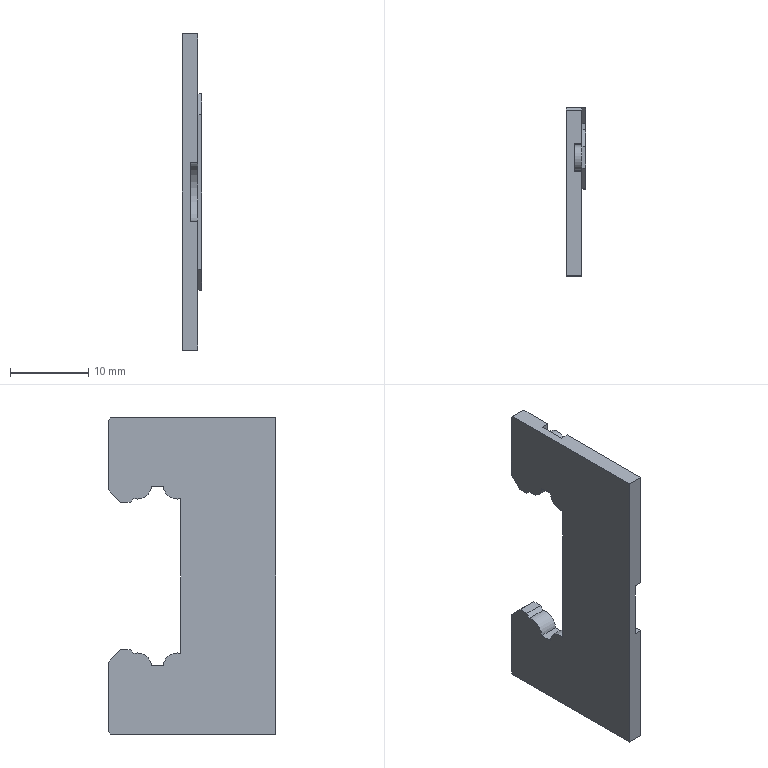Component | NX | SLIDER_1_CLAMP_PLATE | 1 solid | 64 faces | volume 1304 mm3 | plane 55 | cylinder 9 | commonest cylinder face diameters 3.5 x6 3.2 x2 7.5 x1